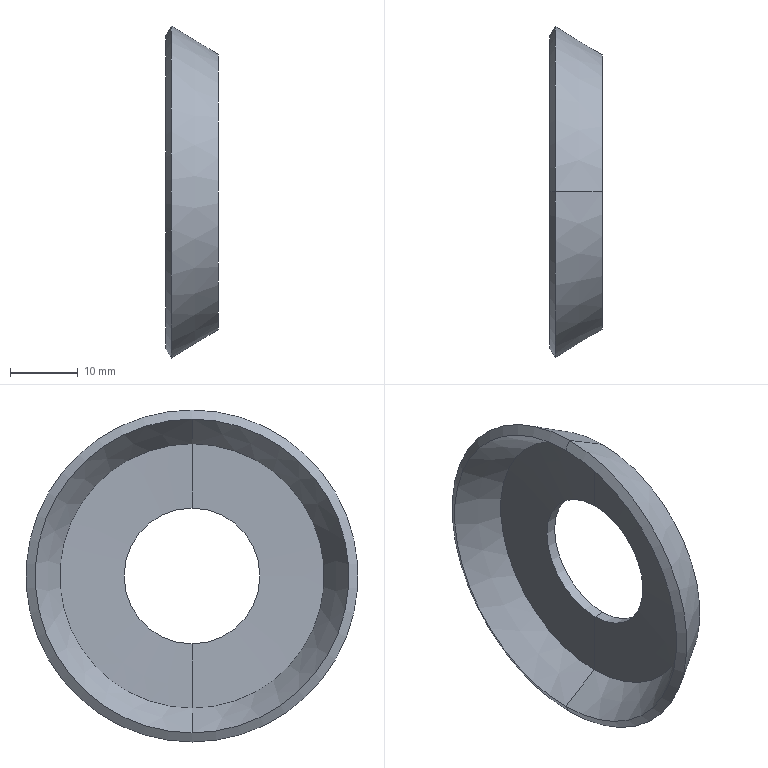Component | SolidWorks | RoundNutLockingWasher15-1 | 1 solid | 11 faces | box 7.71 x 48.93 x 48.93 mm | volume 3191 mm3 | cone 8 | cylinder 2 | plane 1 | commonest cylinder face diameters 20.011 x2
build123d program:
from build123d import *


with BuildPart() as part:
    # Sketch2 → Revolve1 (revolve)
    with BuildSketch(Plane(origin=(0, 0, 0), x_dir=(0, 0, -1), z_dir=(1, 0, 0)), mode=Mode.PRIVATE) as revolve1_sk:
        Polygon((9, 79.719), (3.04, 83.338), (3.857, 84.683), (10.75, 80.498), (10.75, 70.225), (9.15, 70.225), align=None)
    revolve(revolve1_sk.sketch.rotate(Axis((0, 60.219, 215.048), (0, 0, -1)), 90), axis=Axis((0, 60.219, 215.048), (0, 0, -1)))


solid = part.part

# Placed as in the assembly
solid = solid.moved(Location((-196.75, 0, 0), (0, -90, 0)))
STEP:
#1=CARTESIAN_POINT('',(-7.392,2.371,-0.7677));
#2=VERTEX_POINT('',#1);
#3=CARTESIAN_POINT('',(-7.392,2.371,0.7677));
#4=VERTEX_POINT('',#3);
#5=CARTESIAN_POINT('',(-7.392,2.371,0.));
#6=DIRECTION('',(-1.,0.,0.));
#7=DIRECTION('',(0.,0.,1.));
#8=AXIS2_PLACEMENT_3D('',#5,#6,#7);
#9=CIRCLE('',#8,0.7677);
#10=EDGE_CURVE('',#2,#4,#9,.T.);
#11=ORIENTED_EDGE('',*,*,#10,.F.);
#12=CARTESIAN_POINT('',(-7.626,2.371,-0.9102));
#13=VERTEX_POINT('',#12);
#14=CARTESIAN_POINT('',(-7.626,2.371,-0.9102));
#15=DIRECTION('',(-0.8548,0.,-0.519));
#16=VECTOR('',#15,39.37);
#17=LINE('',#14,#16);
#18=EDGE_CURVE('',#2,#13,#17,.T.);
#19=ORIENTED_EDGE('',*,*,#18,.T.);
#20=CARTESIAN_POINT('',(-7.626,2.371,0.9102));
#21=VERTEX_POINT('',#20);
#22=CARTESIAN_POINT('',(-7.626,2.371,0.));
#23=DIRECTION('',(-1.,0.,0.));
#24=DIRECTION('',(0.,0.,1.));
#25=AXIS2_PLACEMENT_3D('',#22,#23,#24);
#26=CIRCLE('',#25,0.9102);
#27=EDGE_CURVE('',#13,#21,#26,.T.);
#28=ORIENTED_EDGE('',*,*,#27,.T.);
#29=CARTESIAN_POINT('',(-7.626,2.371,0.9102));
#30=DIRECTION('',(-0.8548,0.,0.519));
#31=VECTOR('',#30,39.37);
#32=LINE('',#29,#31);
#33=EDGE_CURVE('',#4,#21,#32,.T.);
#34=ORIENTED_EDGE('',*,*,#33,.F.);
#35=EDGE_LOOP('',(#11,#19,#28,#34));
#36=FACE_OUTER_BOUND('',#35,.T.);
#37=CARTESIAN_POINT('',(-7.626,2.371,0.));
#38=DIRECTION('',(-1.,0.,0.));
#39=DIRECTION('',(0.,0.,1.));
#40=AXIS2_PLACEMENT_3D('',#37,#38,#39);
#41=CONICAL_SURFACE('',#40,0.9102,0.5457);
#42=ADVANCED_FACE('',(#36),#41,.F.);
#43=CARTESIAN_POINT('',(-7.626,2.371,0.));
#44=DIRECTION('',(-1.,0.,0.));
#45=DIRECTION('',(0.,0.,1.));
#46=AXIS2_PLACEMENT_3D('',#43,#44,#45);
#47=CIRCLE('',#46,0.9102);
#48=EDGE_CURVE('',#21,#13,#47,.T.);
#49=ORIENTED_EDGE('',*,*,#48,.F.);
#50=CARTESIAN_POINT('',(-7.594,2.371,0.9632));
#51=VERTEX_POINT('',#50);
#52=CARTESIAN_POINT('',(-7.594,2.371,0.9632));
#53=DIRECTION('',(0.519,0.,0.8548));
#54=VECTOR('',#53,39.37);
#55=LINE('',#52,#54);
#56=EDGE_CURVE('',#21,#51,#55,.T.);
#57=ORIENTED_EDGE('',*,*,#56,.T.);
#58=CARTESIAN_POINT('',(-7.594,2.371,-0.9632));
#59=VERTEX_POINT('',#58);
#60=CARTESIAN_POINT('',(-7.594,2.371,0.));
#61=DIRECTION('',(-1.,0.,0.));
#62=DIRECTION('',(0.,0.,1.));
#63=AXIS2_PLACEMENT_3D('',#60,#61,#62);
#64=CIRCLE('',#63,0.9632);
#65=EDGE_CURVE('',#51,#59,#64,.T.);
#66=ORIENTED_EDGE('',*,*,#65,.T.);
#67=CARTESIAN_POINT('',(-7.594,2.371,-0.9632));
#68=DIRECTION('',(0.519,0.,-0.8548));
#69=VECTOR('',#68,39.37);
#70=LINE('',#67,#69);
#71=EDGE_CURVE('',#13,#59,#70,.T.);
#72=ORIENTED_EDGE('',*,*,#71,.F.);
#73=EDGE_LOOP('',(#49,#57,#66,#72));
#74=FACE_OUTER_BOUND('',#73,.T.);
#75=CARTESIAN_POINT('',(-7.594,2.371,0.));
#76=DIRECTION('',(1.,0.,0.));
#77=DIRECTION('',(0.,0.,-1.));
#78=AXIS2_PLACEMENT_3D('',#75,#76,#77);
#79=CONICAL_SURFACE('',#78,0.9632,1.025);
#80=ADVANCED_FACE('',(#74),#79,.T.);
#81=CARTESIAN_POINT('',(-7.323,2.371,0.7984));
#82=VERTEX_POINT('',#81);
#83=CARTESIAN_POINT('',(-7.323,2.371,-0.7984));
#84=VERTEX_POINT('',#83);
#85=CARTESIAN_POINT('',(-7.323,2.371,0.));
#86=DIRECTION('',(-1.,0.,0.));
#87=DIRECTION('',(0.,0.,1.));
#88=AXIS2_PLACEMENT_3D('',#85,#86,#87);
#89=CIRCLE('',#88,0.7984);
#90=EDGE_CURVE('',#82,#84,#89,.T.);
#91=ORIENTED_EDGE('',*,*,#90,.T.);
#92=CARTESIAN_POINT('',(-7.323,2.371,-0.7984));
#93=DIRECTION('',(-0.8548,0.,-0.519));
#94=VECTOR('',#93,39.37);
#95=LINE('',#92,#94);
#96=EDGE_CURVE('',#84,#59,#95,.T.);
#97=ORIENTED_EDGE('',*,*,#96,.T.);
#98=ORIENTED_EDGE('',*,*,#65,.F.);
#99=CARTESIAN_POINT('',(-7.323,2.371,0.7984));
#100=DIRECTION('',(-0.8548,0.,0.519));
#101=VECTOR('',#100,39.37);
#102=LINE('',#99,#101);
#103=EDGE_CURVE('',#82,#51,#102,.T.);
#104=ORIENTED_EDGE('',*,*,#103,.F.);
#105=EDGE_LOOP('',(#91,#97,#98,#104));
#106=FACE_OUTER_BOUND('',#105,.T.);
#107=CARTESIAN_POINT('',(-7.323,2.371,0.));
#108=DIRECTION('',(-1.,0.,0.));
#109=DIRECTION('',(0.,0.,1.));
#110=AXIS2_PLACEMENT_3D('',#107,#108,#109);
#111=CONICAL_SURFACE('',#110,0.7984,0.5457);
#112=ADVANCED_FACE('',(#106),#111,.T.);
#113=CARTESIAN_POINT('',(-7.323,2.371,-0.3939));
#114=VERTEX_POINT('',#113);
#115=CARTESIAN_POINT('',(-7.323,2.371,0.3939));
#116=VERTEX_POINT('',#115);
#117=CARTESIAN_POINT('',(-7.323,2.371,0.));
#118=DIRECTION('',(-1.,0.,0.));
#119=DIRECTION('',(0.,0.,1.));
#120=AXIS2_PLACEMENT_3D('',#117,#118,#119);
#121=CIRCLE('',#120,0.3939);
#122=EDGE_CURVE('',#114,#116,#121,.T.);
#123=ORIENTED_EDGE('',*,*,#122,.F.);
#124=CARTESIAN_POINT('',(-7.386,2.371,-0.3939));
#125=VERTEX_POINT('',#124);
#126=CARTESIAN_POINT('',(-16.213,2.371,-0.3939));
#127=DIRECTION('',(-1.,0.,0.));
#128=VECTOR('',#127,39.37);
#129=LINE('',#126,#128);
#130=EDGE_CURVE('',#114,#125,#129,.T.);
#131=ORIENTED_EDGE('',*,*,#130,.T.);
#132=CARTESIAN_POINT('',(-7.386,2.371,0.3939));
#133=VERTEX_POINT('',#132);
#134=CARTESIAN_POINT('',(-7.386,2.371,0.));
#135=DIRECTION('',(-1.,0.,0.));
#136=DIRECTION('',(0.,0.,1.));
#137=AXIS2_PLACEMENT_3D('',#134,#135,#136);
#138=CIRCLE('',#137,0.3939);
#139=EDGE_CURVE('',#125,#133,#138,.T.);
#140=ORIENTED_EDGE('',*,*,#139,.T.);
#141=CARTESIAN_POINT('',(-16.213,2.371,0.3939));
#142=DIRECTION('',(-1.,0.,0.));
#143=VECTOR('',#142,39.37);
#144=LINE('',#141,#143);
#145=EDGE_CURVE('',#116,#133,#144,.T.);
#146=ORIENTED_EDGE('',*,*,#145,.F.);
#147=EDGE_LOOP('',(#123,#131,#140,#146));
#148=FACE_OUTER_BOUND('',#147,.T.);
#149=CARTESIAN_POINT('',(-16.213,2.371,0.));
#150=DIRECTION('',(-1.,0.,0.));
#151=DIRECTION('',(0.,0.,1.));
#152=AXIS2_PLACEMENT_3D('',#149,#150,#151);
#153=CYLINDRICAL_SURFACE('',#152,0.3939);
#154=ADVANCED_FACE('',(#148),#153,.F.);
#155=ORIENTED_EDGE('',*,*,#139,.F.);
#156=CARTESIAN_POINT('',(-7.392,2.371,-0.7677));
#157=DIRECTION('',(-0.0158,0.,-0.9999));
#158=VECTOR('',#157,39.37);
#159=LINE('',#156,#158);
#160=EDGE_CURVE('',#125,#2,#159,.T.);
#161=ORIENTED_EDGE('',*,*,#160,.T.);
#162=ORIENTED_EDGE('',*,*,#10,.T.);
#163=CARTESIAN_POINT('',(-7.392,2.371,0.7677));
#164=DIRECTION('',(-0.0158,0.,0.9999));
#165=VECTOR('',#164,39.37);
#166=LINE('',#163,#165);
#167=EDGE_CURVE('',#133,#4,#166,.T.);
#168=ORIENTED_EDGE('',*,*,#167,.F.);
#169=EDGE_LOOP('',(#155,#161,#162,#168));
#170=FACE_OUTER_BOUND('',#169,.T.);
#171=CARTESIAN_POINT('',(-7.392,2.371,0.));
#172=DIRECTION('',(-1.,0.,0.));
#173=DIRECTION('',(0.,0.,1.));
#174=AXIS2_PLACEMENT_3D('',#171,#172,#173);
#175=CONICAL_SURFACE('',#174,0.7677,1.555);
#176=ADVANCED_FACE('',(#170),#175,.F.);
#177=ORIENTED_EDGE('',*,*,#160,.F.);
#178=CARTESIAN_POINT('',(-7.386,2.371,0.));
#179=DIRECTION('',(-1.,0.,0.));
#180=DIRECTION('',(0.,0.,1.));
#181=AXIS2_PLACEMENT_3D('',#178,#179,#180);
#182=CIRCLE('',#181,0.3939);
#183=EDGE_CURVE('',#133,#125,#182,.T.);
#184=ORIENTED_EDGE('',*,*,#183,.F.);
#185=ORIENTED_EDGE('',*,*,#167,.T.);
#186=CARTESIAN_POINT('',(-7.392,2.371,0.));
#187=DIRECTION('',(-1.,0.,0.));
#188=DIRECTION('',(0.,0.,1.));
#189=AXIS2_PLACEMENT_3D('',#186,#187,#188);
#190=CIRCLE('',#189,0.7677);
#191=EDGE_CURVE('',#4,#2,#190,.T.);
#192=ORIENTED_EDGE('',*,*,#191,.T.);
#193=EDGE_LOOP('',(#177,#184,#185,#192));
#194=FACE_OUTER_BOUND('',#193,.T.);
#195=CARTESIAN_POINT('',(-7.392,2.371,0.));
#196=DIRECTION('',(-1.,0.,0.));
#197=DIRECTION('',(0.,0.,1.));
#198=AXIS2_PLACEMENT_3D('',#195,#196,#197);
#199=CONICAL_SURFACE('',#198,0.7677,1.555);
#200=ADVANCED_FACE('',(#194),#199,.F.);
#201=ORIENTED_EDGE('',*,*,#130,.F.);
#202=CARTESIAN_POINT('',(-7.323,2.371,0.));
#203=DIRECTION('',(-1.,0.,0.));
#204=DIRECTION('',(0.,0.,1.));
#205=AXIS2_PLACEMENT_3D('',#202,#203,#204);
#206=CIRCLE('',#205,0.3939);
#207=EDGE_CURVE('',#116,#114,#206,.T.);
#208=ORIENTED_EDGE('',*,*,#207,.F.);
#209=ORIENTED_EDGE('',*,*,#145,.T.);
#210=ORIENTED_EDGE('',*,*,#183,.T.);
#211=EDGE_LOOP('',(#201,#208,#209,#210));
#212=FACE_OUTER_BOUND('',#211,.T.);
#213=CARTESIAN_POINT('',(-16.213,2.371,0.));
#214=DIRECTION('',(-1.,0.,0.));
#215=DIRECTION('',(0.,0.,1.));
#216=AXIS2_PLACEMENT_3D('',#213,#214,#215);
#217=CYLINDRICAL_SURFACE('',#216,0.3939);
#218=ADVANCED_FACE('',(#212),#217,.F.);
#219=ORIENTED_EDGE('',*,*,#90,.F.);
#220=CARTESIAN_POINT('',(-7.323,2.371,0.));
#221=DIRECTION('',(-1.,0.,0.));
#222=DIRECTION('',(0.,0.,1.));
#223=AXIS2_PLACEMENT_3D('',#220,#221,#222);
#224=CIRCLE('',#223,0.7984);
#225=EDGE_CURVE('',#84,#82,#224,.T.);
#226=ORIENTED_EDGE('',*,*,#225,.F.);
#227=EDGE_LOOP('',(#219,#226));
#228=FACE_OUTER_BOUND('',#227,.T.);
#229=ORIENTED_EDGE('',*,*,#207,.T.);
#230=ORIENTED_EDGE('',*,*,#122,.T.);
#231=EDGE_LOOP('',(#229,#230));
#232=FACE_BOUND('',#231,.T.);
#233=CARTESIAN_POINT('',(-7.323,3.169,0.));
#234=DIRECTION('',(-1.,0.,0.));
#235=DIRECTION('',(0.,0.,1.));
#236=AXIS2_PLACEMENT_3D('',#233,#234,#235);
#237=PLANE('',#236);
#238=ADVANCED_FACE('',(#228,#232),#237,.F.);
#239=ORIENTED_EDGE('',*,*,#96,.F.);
#240=ORIENTED_EDGE('',*,*,#225,.T.);
#241=ORIENTED_EDGE('',*,*,#103,.T.);
#242=CARTESIAN_POINT('',(-7.594,2.371,0.));
#243=DIRECTION('',(-1.,0.,0.));
#244=DIRECTION('',(0.,0.,1.));
#245=AXIS2_PLACEMENT_3D('',#242,#243,#244);
#246=CIRCLE('',#245,0.9632);
#247=EDGE_CURVE('',#59,#51,#246,.T.);
#248=ORIENTED_EDGE('',*,*,#247,.F.);
#249=EDGE_LOOP('',(#239,#240,#241,#248));
#250=FACE_OUTER_BOUND('',#249,.T.);
#251=CARTESIAN_POINT('',(-7.323,2.371,0.));
#252=DIRECTION('',(-1.,0.,0.));
#253=DIRECTION('',(0.,0.,1.));
#254=AXIS2_PLACEMENT_3D('',#251,#252,#253);
#255=CONICAL_SURFACE('',#254,0.7984,0.5457);
#256=ADVANCED_FACE('',(#250),#255,.T.);
#257=ORIENTED_EDGE('',*,*,#56,.F.);
#258=ORIENTED_EDGE('',*,*,#27,.F.);
#259=ORIENTED_EDGE('',*,*,#71,.T.);
#260=ORIENTED_EDGE('',*,*,#247,.T.);
#261=EDGE_LOOP('',(#257,#258,#259,#260));
#262=FACE_OUTER_BOUND('',#261,.T.);
#263=CARTESIAN_POINT('',(-7.594,2.371,0.));
#264=DIRECTION('',(1.,0.,0.));
#265=DIRECTION('',(0.,0.,-1.));
#266=AXIS2_PLACEMENT_3D('',#263,#264,#265);
#267=CONICAL_SURFACE('',#266,0.9632,1.025);
#268=ADVANCED_FACE('',(#262),#267,.T.);
#269=ORIENTED_EDGE('',*,*,#18,.F.);
#270=ORIENTED_EDGE('',*,*,#191,.F.);
#271=ORIENTED_EDGE('',*,*,#33,.T.);
#272=ORIENTED_EDGE('',*,*,#48,.T.);
#273=EDGE_LOOP('',(#269,#270,#271,#272));
#274=FACE_OUTER_BOUND('',#273,.T.);
#275=CARTESIAN_POINT('',(-7.626,2.371,0.));
#276=DIRECTION('',(-1.,0.,0.));
#277=DIRECTION('',(0.,0.,1.));
#278=AXIS2_PLACEMENT_3D('',#275,#276,#277);
#279=CONICAL_SURFACE('',#278,0.9102,0.5457);
#280=ADVANCED_FACE('',(#274),#279,.F.);
#281=CLOSED_SHELL('',(#42,#80,#112,#154,#176,#200,#218,#238,#256,#268,#280));
#282=MANIFOLD_SOLID_BREP('',#281);
#283=CARTESIAN_POINT('',(0.,0.,0.));
#284=DIRECTION('',(0.,0.,1.));
#285=DIRECTION('',(1.,0.,0.));
#286=AXIS2_PLACEMENT_3D('',#283,#284,#285);
#287=(LENGTH_UNIT()NAMED_UNIT(*)SI_UNIT($,.METRE.));
#288=LENGTH_MEASURE_WITH_UNIT(LENGTH_MEASURE(0.0254),#287);
#289=DIMENSIONAL_EXPONENTS(1.,0.,0.,0.,0.,0.,0.);
#290=(CONVERSION_BASED_UNIT('',#288)LENGTH_UNIT()NAMED_UNIT(#289));
#291=UNCERTAINTY_MEASURE_WITH_UNIT(LENGTH_MEASURE(0.00001),#290,'','');
#292=(NAMED_UNIT(*)PLANE_ANGLE_UNIT()SI_UNIT($,.RADIAN.));
#293=(NAMED_UNIT(*)SI_UNIT($,.STERADIAN.)SOLID_ANGLE_UNIT());
#294=(GEOMETRIC_REPRESENTATION_CONTEXT(3)GLOBAL_UNCERTAINTY_ASSIGNED_CONTEXT((#291))GLOBAL_UNIT_ASSIGNED_CONTEXT((#290,#292,#293))REPRESENTATION_CONTEXT('',''));
#295=ADVANCED_BREP_SHAPE_REPRESENTATION('',(#282,#286),#294);
#296=COLOUR_RGB('',0.7922,0.8196,0.9333);
#297=FILL_AREA_STYLE_COLOUR('',#296);
#298=FILL_AREA_STYLE('',(#297));
#299=SURFACE_STYLE_FILL_AREA(#298);
#300=SURFACE_SIDE_STYLE('',(#299));
#301=SURFACE_STYLE_USAGE(.BOTH.,#300);
#302=PRESENTATION_STYLE_ASSIGNMENT((#301));
#303=STYLED_ITEM('',(#302),#282);
#304=PRESENTATION_LAYER_ASSIGNMENT('','',(#303));
#305=(LENGTH_UNIT()NAMED_UNIT(*)SI_UNIT($,.METRE.));
#306=LENGTH_MEASURE_WITH_UNIT(LENGTH_MEASURE(0.0254),#305);
#307=DIMENSIONAL_EXPONENTS(1.,0.,0.,0.,0.,0.,0.);
#308=(CONVERSION_BASED_UNIT('',#306)LENGTH_UNIT()NAMED_UNIT(#307));
#309=UNCERTAINTY_MEASURE_WITH_UNIT(LENGTH_MEASURE(0.00001),#308,'','');
#310=(NAMED_UNIT(*)PLANE_ANGLE_UNIT()SI_UNIT($,.RADIAN.));
#311=(NAMED_UNIT(*)SI_UNIT($,.STERADIAN.)SOLID_ANGLE_UNIT());
#312=(GEOMETRIC_REPRESENTATION_CONTEXT(3)GLOBAL_UNCERTAINTY_ASSIGNED_CONTEXT((#309))GLOBAL_UNIT_ASSIGNED_CONTEXT((#308,#310,#311))REPRESENTATION_CONTEXT('',''));
#313=MECHANICAL_DESIGN_GEOMETRIC_PRESENTATION_REPRESENTATION('',(#303),#312);